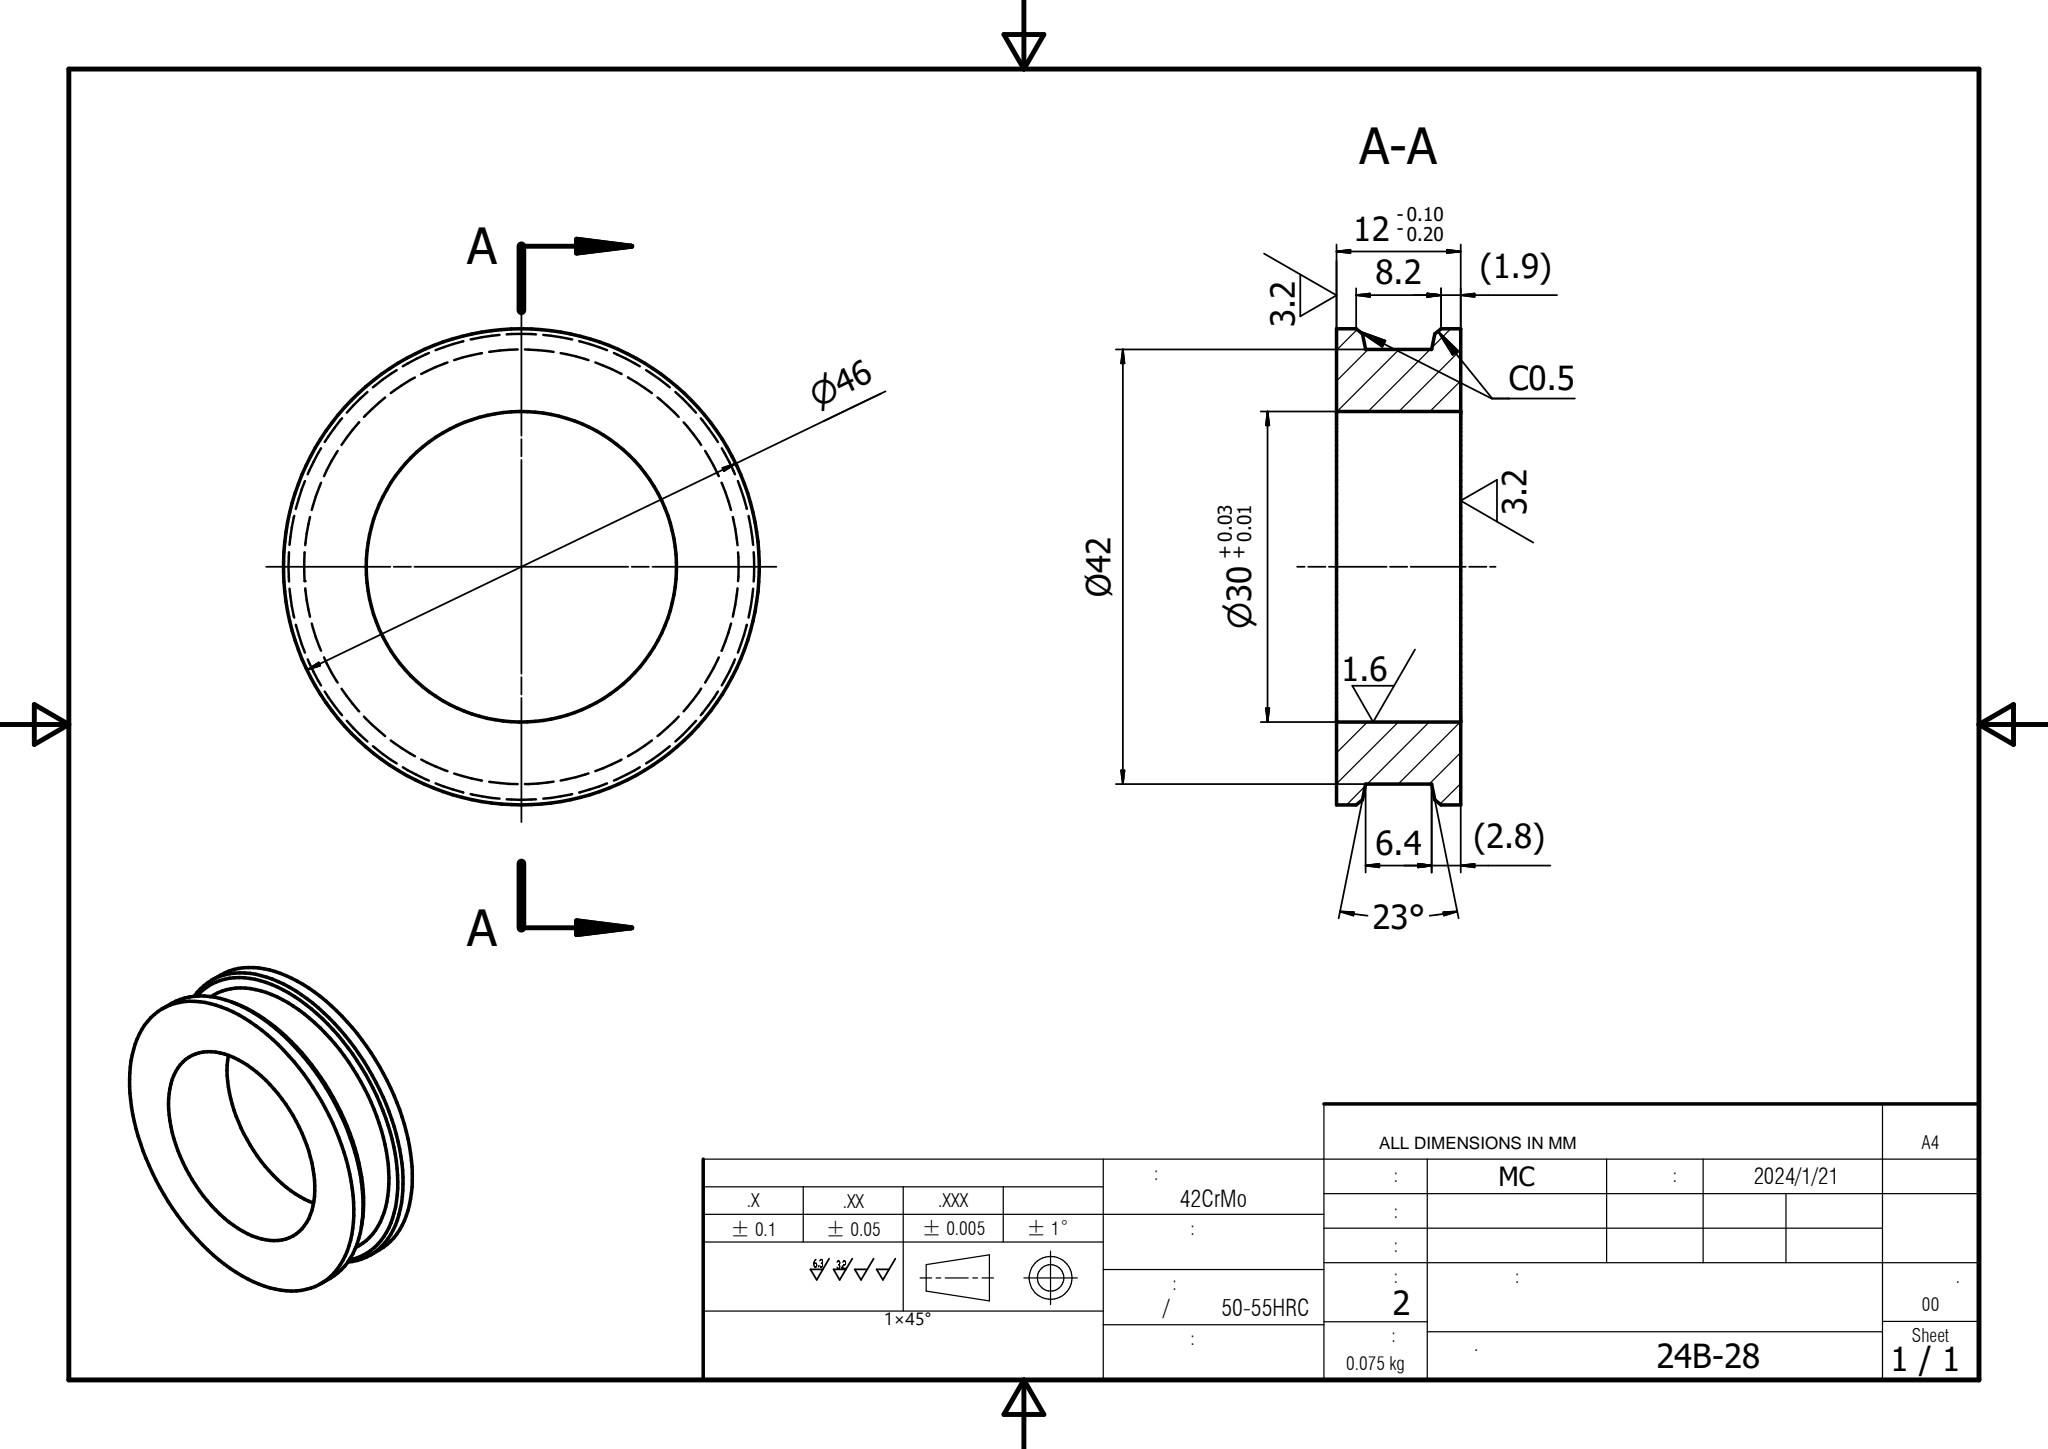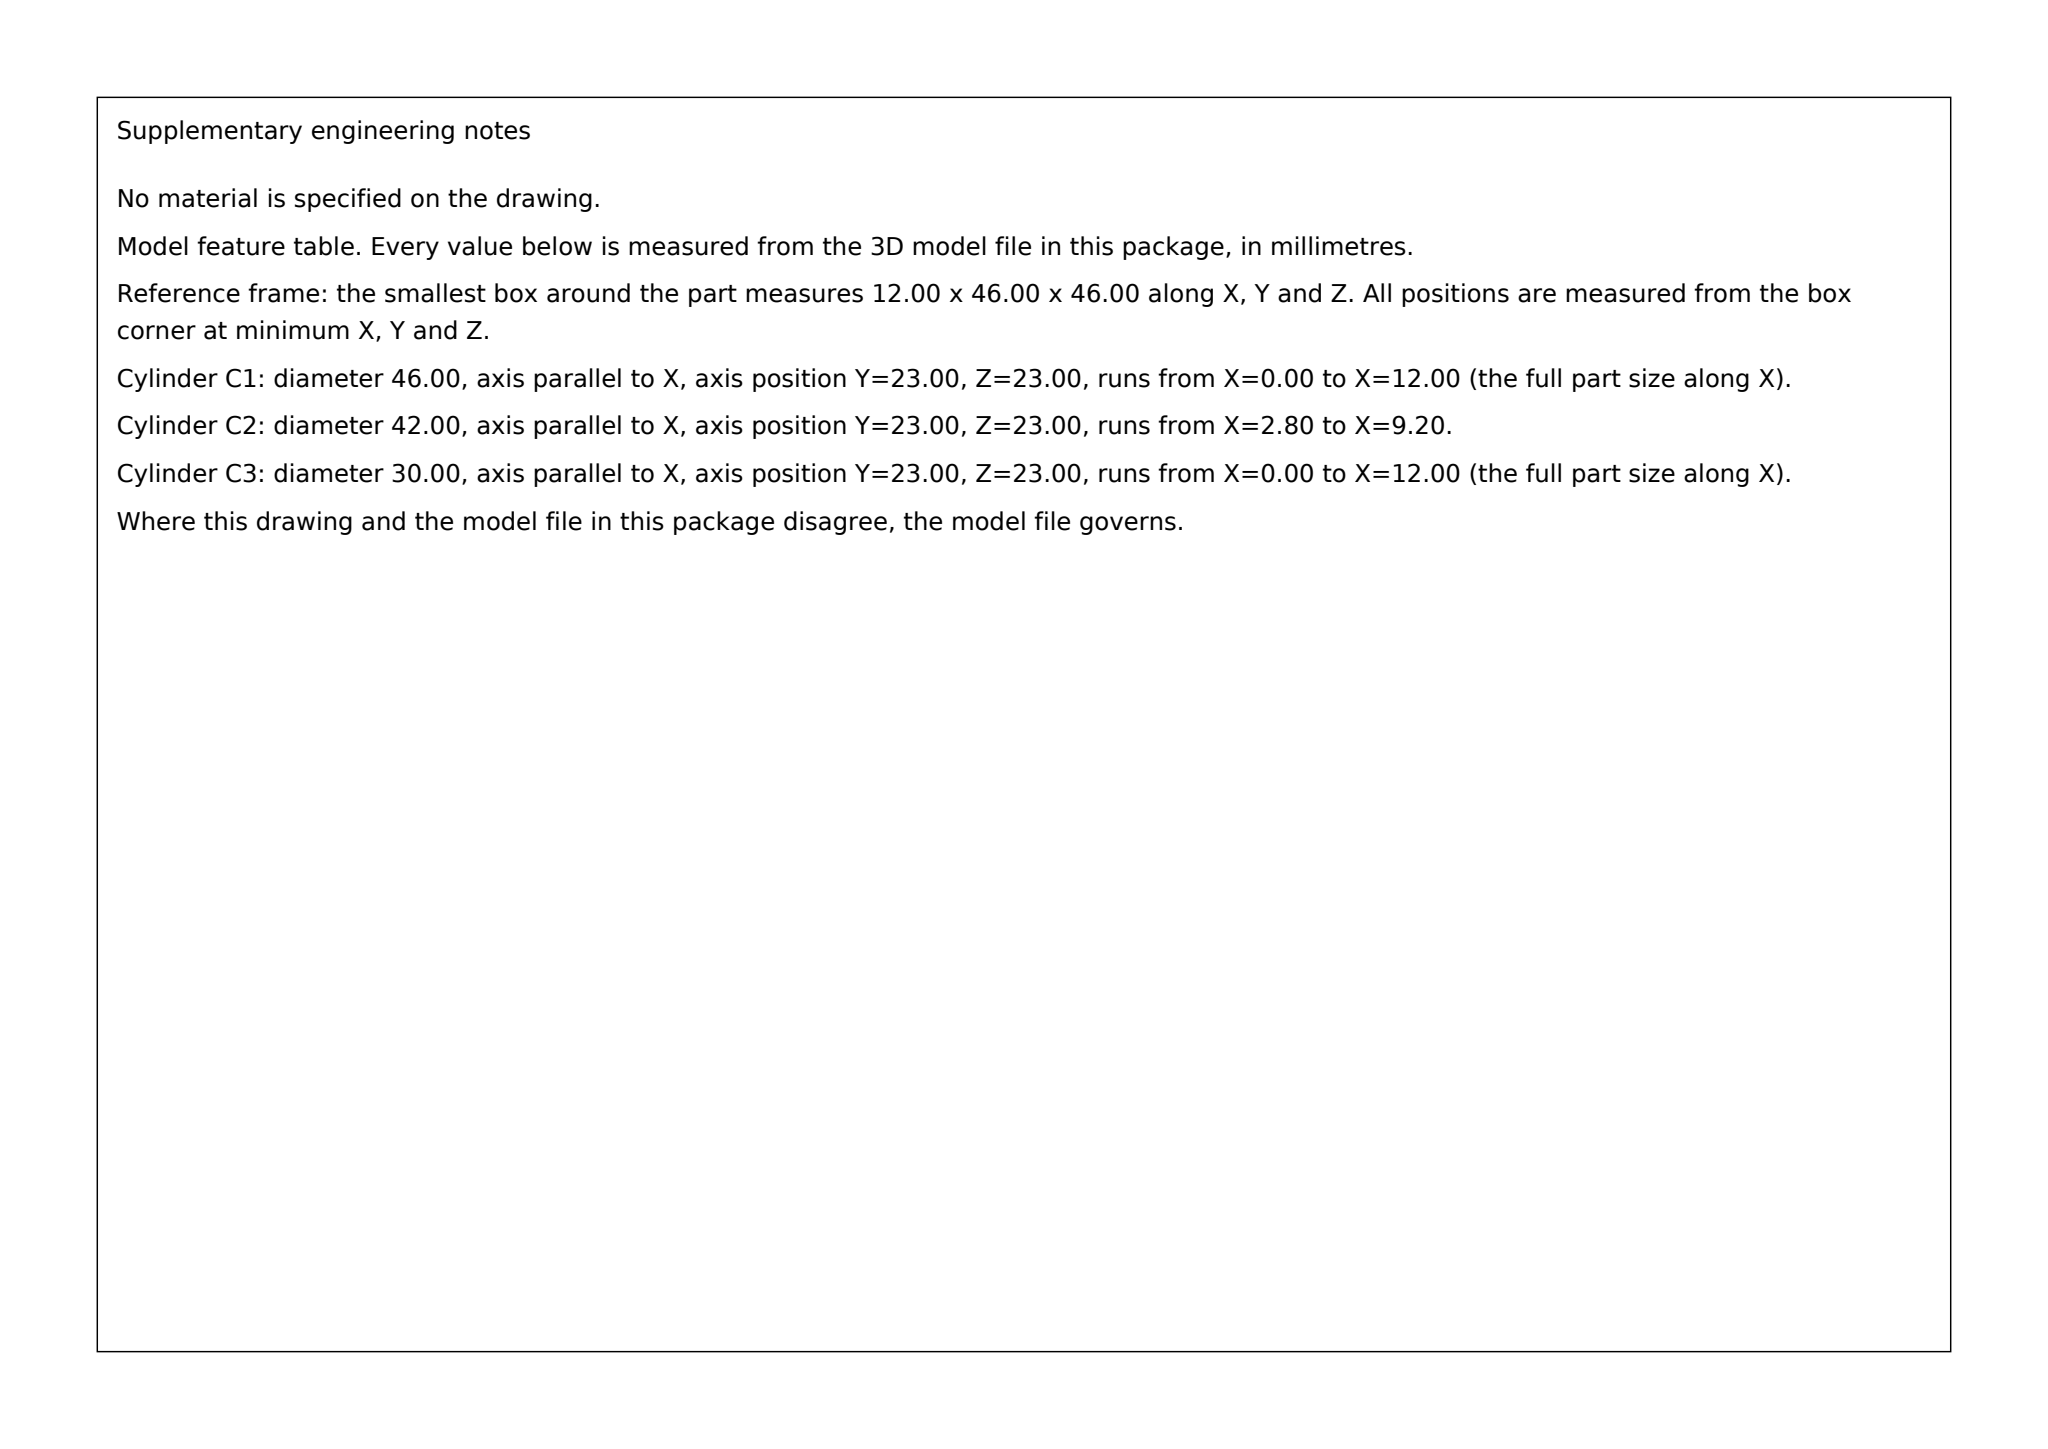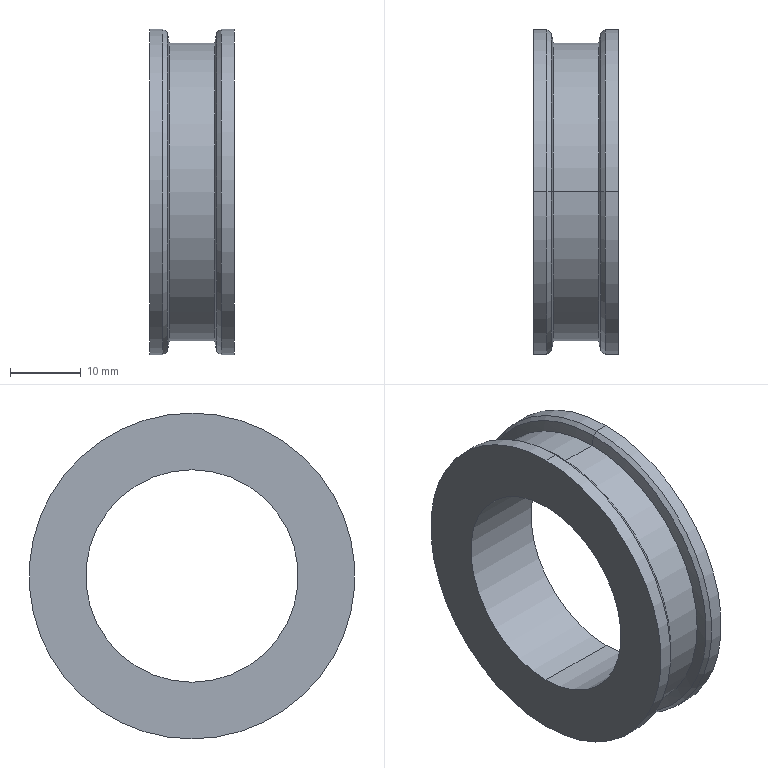Part | SolidWorks | mm | material 42CrMo | 1 solid | 18 faces | box 12 x 46 x 46 mm | volume 9544 mm3 | cylinder 8 | cone 8 | plane 2 | commonest cylinder face diameters 46 x4 30 x2 42 x2
STEP:
#1=CARTESIAN_POINT('',(12.,0.,-15.));
#2=VERTEX_POINT('',#1);
#3=CARTESIAN_POINT('',(12.,0.,15.));
#4=VERTEX_POINT('',#3);
#5=CARTESIAN_POINT('',(12.,0.,0.));
#6=DIRECTION('',(-1.,0.,0.));
#7=DIRECTION('',(0.,0.,1.));
#8=AXIS2_PLACEMENT_3D('',#5,#6,#7);
#9=CIRCLE('',#8,15.);
#10=EDGE_CURVE('',#2,#4,#9,.T.);
#11=ORIENTED_EDGE('',*,*,#10,.F.);
#12=CARTESIAN_POINT('',(0.,0.,-15.));
#13=VERTEX_POINT('',#12);
#14=CARTESIAN_POINT('',(12.,0.,-15.));
#15=DIRECTION('',(-1.,0.,0.));
#16=VECTOR('',#15,1000.);
#17=LINE('',#14,#16);
#18=EDGE_CURVE('',#2,#13,#17,.T.);
#19=ORIENTED_EDGE('',*,*,#18,.T.);
#20=CARTESIAN_POINT('',(0.,0.,15.));
#21=VERTEX_POINT('',#20);
#22=CARTESIAN_POINT('',(0.,0.,0.));
#23=DIRECTION('',(1.,0.,0.));
#24=DIRECTION('',(0.,0.,1.));
#25=AXIS2_PLACEMENT_3D('',#22,#23,#24);
#26=CIRCLE('',#25,15.);
#27=EDGE_CURVE('',#21,#13,#26,.T.);
#28=ORIENTED_EDGE('',*,*,#27,.F.);
#29=CARTESIAN_POINT('',(12.,0.,15.));
#30=DIRECTION('',(-1.,0.,0.));
#31=VECTOR('',#30,1000.);
#32=LINE('',#29,#31);
#33=EDGE_CURVE('',#4,#21,#32,.T.);
#34=ORIENTED_EDGE('',*,*,#33,.F.);
#35=EDGE_LOOP('',(#11,#19,#28,#34));
#36=FACE_OUTER_BOUND('',#35,.T.);
#37=CARTESIAN_POINT('',(12.,0.,0.));
#38=DIRECTION('',(-1.,0.,0.));
#39=DIRECTION('',(0.,0.,1.));
#40=AXIS2_PLACEMENT_3D('',#37,#38,#39);
#41=CYLINDRICAL_SURFACE('',#40,15.);
#42=ADVANCED_FACE('',(#36),#41,.F.);
#43=CARTESIAN_POINT('',(10.1,0.,-23.));
#44=VERTEX_POINT('',#43);
#45=CARTESIAN_POINT('',(10.1,0.,23.));
#46=VERTEX_POINT('',#45);
#47=CARTESIAN_POINT('',(10.1,0.,0.));
#48=DIRECTION('',(1.,0.,0.));
#49=DIRECTION('',(0.,0.,-1.));
#50=AXIS2_PLACEMENT_3D('',#47,#48,#49);
#51=CIRCLE('',#50,23.);
#52=EDGE_CURVE('',#44,#46,#51,.T.);
#53=ORIENTED_EDGE('',*,*,#52,.T.);
#54=CARTESIAN_POINT('',(12.,0.,23.));
#55=VERTEX_POINT('',#54);
#56=CARTESIAN_POINT('',(0.,0.,23.));
#57=DIRECTION('',(1.,0.,0.));
#58=VECTOR('',#57,1000.);
#59=LINE('',#56,#58);
#60=EDGE_CURVE('',#46,#55,#59,.T.);
#61=ORIENTED_EDGE('',*,*,#60,.T.);
#62=CARTESIAN_POINT('',(12.,0.,-23.));
#63=VERTEX_POINT('',#62);
#64=CARTESIAN_POINT('',(12.,0.,0.));
#65=DIRECTION('',(1.,0.,0.));
#66=DIRECTION('',(0.,0.,-1.));
#67=AXIS2_PLACEMENT_3D('',#64,#65,#66);
#68=CIRCLE('',#67,23.);
#69=EDGE_CURVE('',#63,#55,#68,.T.);
#70=ORIENTED_EDGE('',*,*,#69,.F.);
#71=CARTESIAN_POINT('',(0.,0.,-23.));
#72=DIRECTION('',(1.,0.,0.));
#73=VECTOR('',#72,1000.);
#74=LINE('',#71,#73);
#75=EDGE_CURVE('',#44,#63,#74,.T.);
#76=ORIENTED_EDGE('',*,*,#75,.F.);
#77=EDGE_LOOP('',(#53,#61,#70,#76));
#78=FACE_OUTER_BOUND('',#77,.T.);
#79=CARTESIAN_POINT('',(0.,0.,0.));
#80=DIRECTION('',(1.,0.,0.));
#81=DIRECTION('',(0.,0.,-1.));
#82=AXIS2_PLACEMENT_3D('',#79,#80,#81);
#83=CYLINDRICAL_SURFACE('',#82,23.);
#84=ADVANCED_FACE('',(#78),#83,.T.);
#85=CARTESIAN_POINT('',(0.,0.,-23.));
#86=VERTEX_POINT('',#85);
#87=CARTESIAN_POINT('',(0.,0.,23.));
#88=VERTEX_POINT('',#87);
#89=CARTESIAN_POINT('',(0.,0.,0.));
#90=DIRECTION('',(1.,0.,0.));
#91=DIRECTION('',(0.,0.,-1.));
#92=AXIS2_PLACEMENT_3D('',#89,#90,#91);
#93=CIRCLE('',#92,23.);
#94=EDGE_CURVE('',#86,#88,#93,.T.);
#95=ORIENTED_EDGE('',*,*,#94,.T.);
#96=CARTESIAN_POINT('',(1.9,0.,23.));
#97=VERTEX_POINT('',#96);
#98=CARTESIAN_POINT('',(0.,0.,23.));
#99=DIRECTION('',(1.,0.,0.));
#100=VECTOR('',#99,1000.);
#101=LINE('',#98,#100);
#102=EDGE_CURVE('',#88,#97,#101,.T.);
#103=ORIENTED_EDGE('',*,*,#102,.T.);
#104=CARTESIAN_POINT('',(1.9,0.,-23.));
#105=VERTEX_POINT('',#104);
#106=CARTESIAN_POINT('',(1.9,0.,0.));
#107=DIRECTION('',(-1.,0.,0.));
#108=DIRECTION('',(0.,0.,-1.));
#109=AXIS2_PLACEMENT_3D('',#106,#107,#108);
#110=CIRCLE('',#109,23.);
#111=EDGE_CURVE('',#97,#105,#110,.T.);
#112=ORIENTED_EDGE('',*,*,#111,.T.);
#113=CARTESIAN_POINT('',(0.,0.,-23.));
#114=DIRECTION('',(1.,0.,0.));
#115=VECTOR('',#114,1000.);
#116=LINE('',#113,#115);
#117=EDGE_CURVE('',#86,#105,#116,.T.);
#118=ORIENTED_EDGE('',*,*,#117,.F.);
#119=EDGE_LOOP('',(#95,#103,#112,#118));
#120=FACE_OUTER_BOUND('',#119,.T.);
#121=CARTESIAN_POINT('',(0.,0.,0.));
#122=DIRECTION('',(1.,0.,0.));
#123=DIRECTION('',(0.,0.,-1.));
#124=AXIS2_PLACEMENT_3D('',#121,#122,#123);
#125=CYLINDRICAL_SURFACE('',#124,23.);
#126=ADVANCED_FACE('',(#120),#125,.T.);
#127=CARTESIAN_POINT('',(9.502,0.,-22.51));
#128=VERTEX_POINT('',#127);
#129=CARTESIAN_POINT('',(9.502,0.,22.51));
#130=VERTEX_POINT('',#129);
#131=CARTESIAN_POINT('',(9.502,0.,0.));
#132=DIRECTION('',(1.,0.,-0.));
#133=DIRECTION('',(0.,-1.,0.));
#134=AXIS2_PLACEMENT_3D('',#131,#132,#133);
#135=CIRCLE('',#134,22.51);
#136=EDGE_CURVE('',#128,#130,#135,.T.);
#137=ORIENTED_EDGE('',*,*,#136,.T.);
#138=CARTESIAN_POINT('',(10.1,0.,23.));
#139=DIRECTION('',(0.7733,0.,0.634));
#140=VECTOR('',#139,1000.);
#141=LINE('',#138,#140);
#142=EDGE_CURVE('',#130,#46,#141,.T.);
#143=ORIENTED_EDGE('',*,*,#142,.T.);
#144=ORIENTED_EDGE('',*,*,#52,.F.);
#145=CARTESIAN_POINT('',(10.1,0.,-23.));
#146=DIRECTION('',(0.7733,0.,-0.634));
#147=VECTOR('',#146,1000.);
#148=LINE('',#145,#147);
#149=EDGE_CURVE('',#128,#44,#148,.T.);
#150=ORIENTED_EDGE('',*,*,#149,.F.);
#151=EDGE_LOOP('',(#137,#143,#144,#150));
#152=FACE_OUTER_BOUND('',#151,.T.);
#153=CARTESIAN_POINT('',(10.1,0.,0.));
#154=DIRECTION('',(1.,0.,-0.));
#155=DIRECTION('',(-0.,0.,-1.));
#156=AXIS2_PLACEMENT_3D('',#153,#154,#155);
#157=CONICAL_SURFACE('',#156,23.,0.6867);
#158=ADVANCED_FACE('',(#152),#157,.T.);
#159=CARTESIAN_POINT('',(2.498,0.,22.51));
#160=VERTEX_POINT('',#159);
#161=CARTESIAN_POINT('',(2.498,0.,-22.51));
#162=VERTEX_POINT('',#161);
#163=CARTESIAN_POINT('',(2.498,0.,0.));
#164=DIRECTION('',(-1.,0.,-0.));
#165=DIRECTION('',(-0.,-1.,0.));
#166=AXIS2_PLACEMENT_3D('',#163,#164,#165);
#167=CIRCLE('',#166,22.51);
#168=EDGE_CURVE('',#160,#162,#167,.T.);
#169=ORIENTED_EDGE('',*,*,#168,.T.);
#170=CARTESIAN_POINT('',(1.9,0.,-23.));
#171=DIRECTION('',(-0.7733,0.,-0.634));
#172=VECTOR('',#171,1000.);
#173=LINE('',#170,#172);
#174=EDGE_CURVE('',#162,#105,#173,.T.);
#175=ORIENTED_EDGE('',*,*,#174,.T.);
#176=ORIENTED_EDGE('',*,*,#111,.F.);
#177=CARTESIAN_POINT('',(1.9,0.,23.));
#178=DIRECTION('',(-0.7733,0.,0.634));
#179=VECTOR('',#178,1000.);
#180=LINE('',#177,#179);
#181=EDGE_CURVE('',#160,#97,#180,.T.);
#182=ORIENTED_EDGE('',*,*,#181,.F.);
#183=EDGE_LOOP('',(#169,#175,#176,#182));
#184=FACE_OUTER_BOUND('',#183,.T.);
#185=CARTESIAN_POINT('',(1.9,0.,0.));
#186=DIRECTION('',(-1.,0.,-0.));
#187=DIRECTION('',(-0.,0.,1.));
#188=AXIS2_PLACEMENT_3D('',#185,#186,#187);
#189=CONICAL_SURFACE('',#188,23.,0.6867);
#190=ADVANCED_FACE('',(#184),#189,.T.);
#191=CARTESIAN_POINT('',(9.2,0.,-21.));
#192=VERTEX_POINT('',#191);
#193=CARTESIAN_POINT('',(9.2,0.,21.));
#194=VERTEX_POINT('',#193);
#195=CARTESIAN_POINT('',(9.2,0.,0.));
#196=DIRECTION('',(1.,0.,0.));
#197=DIRECTION('',(0.,1.,0.));
#198=AXIS2_PLACEMENT_3D('',#195,#196,#197);
#199=CIRCLE('',#198,21.);
#200=EDGE_CURVE('',#192,#194,#199,.T.);
#201=ORIENTED_EDGE('',*,*,#200,.T.);
#202=CARTESIAN_POINT('',(9.502,0.,22.51));
#203=DIRECTION('',(0.1961,0.,0.9806));
#204=VECTOR('',#203,1000.);
#205=LINE('',#202,#204);
#206=EDGE_CURVE('',#194,#130,#205,.T.);
#207=ORIENTED_EDGE('',*,*,#206,.T.);
#208=ORIENTED_EDGE('',*,*,#136,.F.);
#209=CARTESIAN_POINT('',(9.502,0.,-22.51));
#210=DIRECTION('',(0.1961,0.,-0.9806));
#211=VECTOR('',#210,1000.);
#212=LINE('',#209,#211);
#213=EDGE_CURVE('',#192,#128,#212,.T.);
#214=ORIENTED_EDGE('',*,*,#213,.F.);
#215=EDGE_LOOP('',(#201,#207,#208,#214));
#216=FACE_OUTER_BOUND('',#215,.T.);
#217=CARTESIAN_POINT('',(9.502,0.,0.));
#218=DIRECTION('',(1.,0.,0.));
#219=DIRECTION('',(0.,0.,-1.));
#220=AXIS2_PLACEMENT_3D('',#217,#218,#219);
#221=CONICAL_SURFACE('',#220,22.51,1.373);
#222=ADVANCED_FACE('',(#216),#221,.T.);
#223=CARTESIAN_POINT('',(2.8,0.,21.));
#224=VERTEX_POINT('',#223);
#225=CARTESIAN_POINT('',(2.8,0.,-21.));
#226=VERTEX_POINT('',#225);
#227=CARTESIAN_POINT('',(2.8,0.,0.));
#228=DIRECTION('',(-1.,0.,0.));
#229=DIRECTION('',(0.,1.,0.));
#230=AXIS2_PLACEMENT_3D('',#227,#228,#229);
#231=CIRCLE('',#230,21.);
#232=EDGE_CURVE('',#224,#226,#231,.T.);
#233=ORIENTED_EDGE('',*,*,#232,.T.);
#234=CARTESIAN_POINT('',(2.498,0.,-22.51));
#235=DIRECTION('',(-0.1961,0.,-0.9806));
#236=VECTOR('',#235,1000.);
#237=LINE('',#234,#236);
#238=EDGE_CURVE('',#226,#162,#237,.T.);
#239=ORIENTED_EDGE('',*,*,#238,.T.);
#240=ORIENTED_EDGE('',*,*,#168,.F.);
#241=CARTESIAN_POINT('',(2.498,0.,22.51));
#242=DIRECTION('',(-0.1961,0.,0.9806));
#243=VECTOR('',#242,1000.);
#244=LINE('',#241,#243);
#245=EDGE_CURVE('',#224,#160,#244,.T.);
#246=ORIENTED_EDGE('',*,*,#245,.F.);
#247=EDGE_LOOP('',(#233,#239,#240,#246));
#248=FACE_OUTER_BOUND('',#247,.T.);
#249=CARTESIAN_POINT('',(2.498,0.,0.));
#250=DIRECTION('',(-1.,0.,0.));
#251=DIRECTION('',(0.,0.,1.));
#252=AXIS2_PLACEMENT_3D('',#249,#250,#251);
#253=CONICAL_SURFACE('',#252,22.51,1.373);
#254=ADVANCED_FACE('',(#248),#253,.T.);
#255=ORIENTED_EDGE('',*,*,#200,.F.);
#256=CARTESIAN_POINT('',(6.,0.,-21.));
#257=DIRECTION('',(-1.,0.,0.));
#258=VECTOR('',#257,1000.);
#259=LINE('',#256,#258);
#260=EDGE_CURVE('',#192,#226,#259,.T.);
#261=ORIENTED_EDGE('',*,*,#260,.T.);
#262=ORIENTED_EDGE('',*,*,#232,.F.);
#263=CARTESIAN_POINT('',(6.,0.,21.));
#264=DIRECTION('',(-1.,0.,0.));
#265=VECTOR('',#264,1000.);
#266=LINE('',#263,#265);
#267=EDGE_CURVE('',#194,#224,#266,.T.);
#268=ORIENTED_EDGE('',*,*,#267,.F.);
#269=EDGE_LOOP('',(#255,#261,#262,#268));
#270=FACE_OUTER_BOUND('',#269,.T.);
#271=CARTESIAN_POINT('',(6.,0.,0.));
#272=DIRECTION('',(-1.,0.,0.));
#273=DIRECTION('',(0.,0.,1.));
#274=AXIS2_PLACEMENT_3D('',#271,#272,#273);
#275=CYLINDRICAL_SURFACE('',#274,21.);
#276=ADVANCED_FACE('',(#270),#275,.T.);
#277=ORIENTED_EDGE('',*,*,#18,.F.);
#278=CARTESIAN_POINT('',(12.,0.,0.));
#279=DIRECTION('',(-1.,0.,0.));
#280=DIRECTION('',(0.,0.,1.));
#281=AXIS2_PLACEMENT_3D('',#278,#279,#280);
#282=CIRCLE('',#281,15.);
#283=EDGE_CURVE('',#4,#2,#282,.T.);
#284=ORIENTED_EDGE('',*,*,#283,.F.);
#285=ORIENTED_EDGE('',*,*,#33,.T.);
#286=CARTESIAN_POINT('',(0.,0.,0.));
#287=DIRECTION('',(1.,0.,0.));
#288=DIRECTION('',(0.,0.,1.));
#289=AXIS2_PLACEMENT_3D('',#286,#287,#288);
#290=CIRCLE('',#289,15.);
#291=EDGE_CURVE('',#13,#21,#290,.T.);
#292=ORIENTED_EDGE('',*,*,#291,.F.);
#293=EDGE_LOOP('',(#277,#284,#285,#292));
#294=FACE_OUTER_BOUND('',#293,.T.);
#295=CARTESIAN_POINT('',(12.,0.,0.));
#296=DIRECTION('',(-1.,0.,0.));
#297=DIRECTION('',(0.,0.,1.));
#298=AXIS2_PLACEMENT_3D('',#295,#296,#297);
#299=CYLINDRICAL_SURFACE('',#298,15.);
#300=ADVANCED_FACE('',(#294),#299,.F.);
#301=ORIENTED_EDGE('',*,*,#283,.T.);
#302=ORIENTED_EDGE('',*,*,#10,.T.);
#303=EDGE_LOOP('',(#301,#302));
#304=FACE_BOUND('',#303,.T.);
#305=ORIENTED_EDGE('',*,*,#69,.T.);
#306=CARTESIAN_POINT('',(12.,0.,0.));
#307=DIRECTION('',(1.,0.,0.));
#308=DIRECTION('',(0.,0.,-1.));
#309=AXIS2_PLACEMENT_3D('',#306,#307,#308);
#310=CIRCLE('',#309,23.);
#311=EDGE_CURVE('',#55,#63,#310,.T.);
#312=ORIENTED_EDGE('',*,*,#311,.T.);
#313=EDGE_LOOP('',(#305,#312));
#314=FACE_OUTER_BOUND('',#313,.T.);
#315=CARTESIAN_POINT('',(12.,0.,0.));
#316=DIRECTION('',(1.,0.,0.));
#317=DIRECTION('',(0.,0.,-1.));
#318=AXIS2_PLACEMENT_3D('',#315,#316,#317);
#319=PLANE('',#318);
#320=ADVANCED_FACE('',(#304,#314),#319,.T.);
#321=ORIENTED_EDGE('',*,*,#27,.T.);
#322=ORIENTED_EDGE('',*,*,#291,.T.);
#323=EDGE_LOOP('',(#321,#322));
#324=FACE_BOUND('',#323,.T.);
#325=ORIENTED_EDGE('',*,*,#94,.F.);
#326=CARTESIAN_POINT('',(0.,0.,0.));
#327=DIRECTION('',(1.,0.,0.));
#328=DIRECTION('',(0.,0.,-1.));
#329=AXIS2_PLACEMENT_3D('',#326,#327,#328);
#330=CIRCLE('',#329,23.);
#331=EDGE_CURVE('',#88,#86,#330,.T.);
#332=ORIENTED_EDGE('',*,*,#331,.F.);
#333=EDGE_LOOP('',(#325,#332));
#334=FACE_OUTER_BOUND('',#333,.T.);
#335=CARTESIAN_POINT('',(0.,0.,0.));
#336=DIRECTION('',(1.,0.,0.));
#337=DIRECTION('',(0.,0.,-1.));
#338=AXIS2_PLACEMENT_3D('',#335,#336,#337);
#339=PLANE('',#338);
#340=ADVANCED_FACE('',(#324,#334),#339,.F.);
#341=ORIENTED_EDGE('',*,*,#60,.F.);
#342=CARTESIAN_POINT('',(10.1,0.,0.));
#343=DIRECTION('',(1.,0.,0.));
#344=DIRECTION('',(0.,0.,-1.));
#345=AXIS2_PLACEMENT_3D('',#342,#343,#344);
#346=CIRCLE('',#345,23.);
#347=EDGE_CURVE('',#46,#44,#346,.T.);
#348=ORIENTED_EDGE('',*,*,#347,.T.);
#349=ORIENTED_EDGE('',*,*,#75,.T.);
#350=ORIENTED_EDGE('',*,*,#311,.F.);
#351=EDGE_LOOP('',(#341,#348,#349,#350));
#352=FACE_OUTER_BOUND('',#351,.T.);
#353=CARTESIAN_POINT('',(0.,0.,0.));
#354=DIRECTION('',(1.,0.,0.));
#355=DIRECTION('',(0.,0.,-1.));
#356=AXIS2_PLACEMENT_3D('',#353,#354,#355);
#357=CYLINDRICAL_SURFACE('',#356,23.);
#358=ADVANCED_FACE('',(#352),#357,.T.);
#359=ORIENTED_EDGE('',*,*,#102,.F.);
#360=ORIENTED_EDGE('',*,*,#331,.T.);
#361=ORIENTED_EDGE('',*,*,#117,.T.);
#362=CARTESIAN_POINT('',(1.9,0.,0.));
#363=DIRECTION('',(-1.,0.,0.));
#364=DIRECTION('',(0.,0.,-1.));
#365=AXIS2_PLACEMENT_3D('',#362,#363,#364);
#366=CIRCLE('',#365,23.);
#367=EDGE_CURVE('',#105,#97,#366,.T.);
#368=ORIENTED_EDGE('',*,*,#367,.T.);
#369=EDGE_LOOP('',(#359,#360,#361,#368));
#370=FACE_OUTER_BOUND('',#369,.T.);
#371=CARTESIAN_POINT('',(0.,0.,0.));
#372=DIRECTION('',(1.,0.,0.));
#373=DIRECTION('',(0.,0.,-1.));
#374=AXIS2_PLACEMENT_3D('',#371,#372,#373);
#375=CYLINDRICAL_SURFACE('',#374,23.);
#376=ADVANCED_FACE('',(#370),#375,.T.);
#377=ORIENTED_EDGE('',*,*,#142,.F.);
#378=CARTESIAN_POINT('',(9.502,0.,0.));
#379=DIRECTION('',(1.,0.,-0.));
#380=DIRECTION('',(0.,-1.,0.));
#381=AXIS2_PLACEMENT_3D('',#378,#379,#380);
#382=CIRCLE('',#381,22.51);
#383=EDGE_CURVE('',#130,#128,#382,.T.);
#384=ORIENTED_EDGE('',*,*,#383,.T.);
#385=ORIENTED_EDGE('',*,*,#149,.T.);
#386=ORIENTED_EDGE('',*,*,#347,.F.);
#387=EDGE_LOOP('',(#377,#384,#385,#386));
#388=FACE_OUTER_BOUND('',#387,.T.);
#389=CARTESIAN_POINT('',(10.1,0.,0.));
#390=DIRECTION('',(1.,0.,-0.));
#391=DIRECTION('',(-0.,0.,-1.));
#392=AXIS2_PLACEMENT_3D('',#389,#390,#391);
#393=CONICAL_SURFACE('',#392,23.,0.6867);
#394=ADVANCED_FACE('',(#388),#393,.T.);
#395=ORIENTED_EDGE('',*,*,#174,.F.);
#396=CARTESIAN_POINT('',(2.498,0.,0.));
#397=DIRECTION('',(-1.,0.,-0.));
#398=DIRECTION('',(-0.,-1.,0.));
#399=AXIS2_PLACEMENT_3D('',#396,#397,#398);
#400=CIRCLE('',#399,22.51);
#401=EDGE_CURVE('',#162,#160,#400,.T.);
#402=ORIENTED_EDGE('',*,*,#401,.T.);
#403=ORIENTED_EDGE('',*,*,#181,.T.);
#404=ORIENTED_EDGE('',*,*,#367,.F.);
#405=EDGE_LOOP('',(#395,#402,#403,#404));
#406=FACE_OUTER_BOUND('',#405,.T.);
#407=CARTESIAN_POINT('',(1.9,0.,0.));
#408=DIRECTION('',(-1.,0.,-0.));
#409=DIRECTION('',(-0.,0.,1.));
#410=AXIS2_PLACEMENT_3D('',#407,#408,#409);
#411=CONICAL_SURFACE('',#410,23.,0.6867);
#412=ADVANCED_FACE('',(#406),#411,.T.);
#413=ORIENTED_EDGE('',*,*,#206,.F.);
#414=CARTESIAN_POINT('',(9.2,0.,0.));
#415=DIRECTION('',(1.,0.,0.));
#416=DIRECTION('',(0.,1.,0.));
#417=AXIS2_PLACEMENT_3D('',#414,#415,#416);
#418=CIRCLE('',#417,21.);
#419=EDGE_CURVE('',#194,#192,#418,.T.);
#420=ORIENTED_EDGE('',*,*,#419,.T.);
#421=ORIENTED_EDGE('',*,*,#213,.T.);
#422=ORIENTED_EDGE('',*,*,#383,.F.);
#423=EDGE_LOOP('',(#413,#420,#421,#422));
#424=FACE_OUTER_BOUND('',#423,.T.);
#425=CARTESIAN_POINT('',(9.502,0.,0.));
#426=DIRECTION('',(1.,0.,0.));
#427=DIRECTION('',(0.,0.,-1.));
#428=AXIS2_PLACEMENT_3D('',#425,#426,#427);
#429=CONICAL_SURFACE('',#428,22.51,1.373);
#430=ADVANCED_FACE('',(#424),#429,.T.);
#431=ORIENTED_EDGE('',*,*,#238,.F.);
#432=CARTESIAN_POINT('',(2.8,0.,0.));
#433=DIRECTION('',(-1.,0.,0.));
#434=DIRECTION('',(0.,1.,0.));
#435=AXIS2_PLACEMENT_3D('',#432,#433,#434);
#436=CIRCLE('',#435,21.);
#437=EDGE_CURVE('',#226,#224,#436,.T.);
#438=ORIENTED_EDGE('',*,*,#437,.T.);
#439=ORIENTED_EDGE('',*,*,#245,.T.);
#440=ORIENTED_EDGE('',*,*,#401,.F.);
#441=EDGE_LOOP('',(#431,#438,#439,#440));
#442=FACE_OUTER_BOUND('',#441,.T.);
#443=CARTESIAN_POINT('',(2.498,0.,0.));
#444=DIRECTION('',(-1.,0.,0.));
#445=DIRECTION('',(0.,0.,1.));
#446=AXIS2_PLACEMENT_3D('',#443,#444,#445);
#447=CONICAL_SURFACE('',#446,22.51,1.373);
#448=ADVANCED_FACE('',(#442),#447,.T.);
#449=ORIENTED_EDGE('',*,*,#260,.F.);
#450=ORIENTED_EDGE('',*,*,#419,.F.);
#451=ORIENTED_EDGE('',*,*,#267,.T.);
#452=ORIENTED_EDGE('',*,*,#437,.F.);
#453=EDGE_LOOP('',(#449,#450,#451,#452));
#454=FACE_OUTER_BOUND('',#453,.T.);
#455=CARTESIAN_POINT('',(6.,0.,0.));
#456=DIRECTION('',(-1.,0.,0.));
#457=DIRECTION('',(0.,0.,1.));
#458=AXIS2_PLACEMENT_3D('',#455,#456,#457);
#459=CYLINDRICAL_SURFACE('',#458,21.);
#460=ADVANCED_FACE('',(#454),#459,.T.);
#461=CLOSED_SHELL('',(#42,#84,#126,#158,#190,#222,#254,#276,#300,#320,#340,#358,#376,#394,#412,#430,#448,#460));
#462=MANIFOLD_SOLID_BREP('',#461);
#463=CARTESIAN_POINT('',(0.,0.,0.));
#464=DIRECTION('',(0.,0.,1.));
#465=DIRECTION('',(1.,0.,0.));
#466=AXIS2_PLACEMENT_3D('',#463,#464,#465);
#467=(LENGTH_UNIT()NAMED_UNIT(*)SI_UNIT(.MILLI.,.METRE.));
#468=UNCERTAINTY_MEASURE_WITH_UNIT(LENGTH_MEASURE(0.00001),#467,'','');
#469=(NAMED_UNIT(*)PLANE_ANGLE_UNIT()SI_UNIT($,.RADIAN.));
#470=(NAMED_UNIT(*)SI_UNIT($,.STERADIAN.)SOLID_ANGLE_UNIT());
#471=(GEOMETRIC_REPRESENTATION_CONTEXT(3)GLOBAL_UNCERTAINTY_ASSIGNED_CONTEXT((#468))GLOBAL_UNIT_ASSIGNED_CONTEXT((#467,#469,#470))REPRESENTATION_CONTEXT('',''));
#472=ADVANCED_BREP_SHAPE_REPRESENTATION('',(#462,#466),#471);